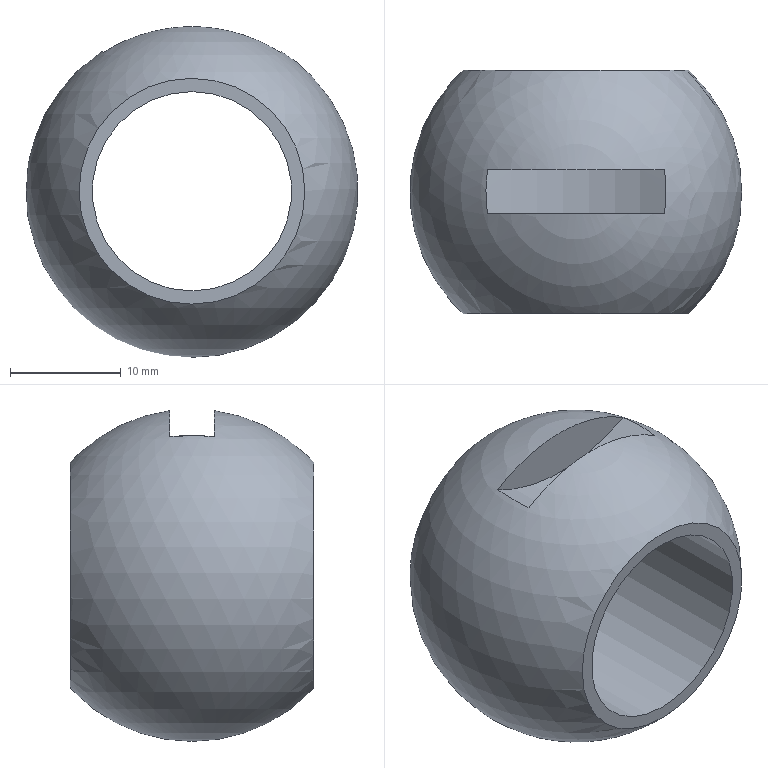Component | NX | VALVE_CORE | 1 solid | 7 faces | box 30 x 22 x 29.87 mm | volume 6970 mm3 | plane 4 | cylinder 2 | sphere 1 | commonest cylinder face diameters 18 x1 33.5 x1
STEP:
#1=CARTESIAN_POINT('',(0.,0.,0.));
#2=DIRECTION('',(0.,0.,1.));
#3=DIRECTION('',(1.,0.,0.));
#4=AXIS2_PLACEMENT_3D('',#1,#2,#3);
#5=CARTESIAN_POINT('',(-7.997,16.,31.532));
#6=VERTEX_POINT('',#5);
#7=CARTESIAN_POINT('',(-7.997,12.,31.532));
#8=VERTEX_POINT('',#7);
#9=CARTESIAN_POINT('',(-7.997,16.,31.532));
#10=CARTESIAN_POINT('',(-8.177,14.667,31.63));
#11=CARTESIAN_POINT('',(-8.177,13.333,31.63));
#12=CARTESIAN_POINT('',(-7.997,12.,31.532));
#13=B_SPLINE_CURVE_WITH_KNOTS('',3,(#9,#10,#11,#12),.UNSPECIFIED.,.F.,.F.,(4,4),(0.,1.),.PIECEWISE_BEZIER_KNOTS.);
#14=CARTESIAN_POINT('',(-0.,14.,19.));
#15=DIRECTION('',(0.,0.,1.));
#16=DIRECTION('',(1.,0.,-0.));
#17=AXIS2_PLACEMENT_3D('',#14,#15,#16);
#18=SPHERICAL_SURFACE('',#17,15.);
#19=CARTESIAN_POINT('',(2.897,0.989));
#20=CARTESIAN_POINT('',(2.904,0.9895));
#21=CARTESIAN_POINT('',(2.919,0.9906));
#22=CARTESIAN_POINT('',(2.941,0.992));
#23=CARTESIAN_POINT('',(2.963,0.9932));
#24=CARTESIAN_POINT('',(2.985,0.9943));
#25=CARTESIAN_POINT('',(3.008,0.9953));
#26=CARTESIAN_POINT('',(3.03,0.9961));
#27=CARTESIAN_POINT('',(3.052,0.9967));
#28=CARTESIAN_POINT('',(3.075,0.9972));
#29=CARTESIAN_POINT('',(3.097,0.9976));
#30=CARTESIAN_POINT('',(3.119,0.9978));
#31=CARTESIAN_POINT('',(3.142,0.9979));
#32=CARTESIAN_POINT('',(3.164,0.9978));
#33=CARTESIAN_POINT('',(3.186,0.9976));
#34=CARTESIAN_POINT('',(3.209,0.9972));
#35=CARTESIAN_POINT('',(3.231,0.9967));
#36=CARTESIAN_POINT('',(3.253,0.9961));
#37=CARTESIAN_POINT('',(3.276,0.9953));
#38=CARTESIAN_POINT('',(3.298,0.9943));
#39=CARTESIAN_POINT('',(3.32,0.9932));
#40=CARTESIAN_POINT('',(3.342,0.992));
#41=CARTESIAN_POINT('',(3.365,0.9906));
#42=CARTESIAN_POINT('',(3.379,0.9895));
#43=CARTESIAN_POINT('',(3.387,0.989));
#44=B_SPLINE_CURVE_WITH_KNOTS('',3,(#19,#20,#21,#22,#23,#24,#25,#26,#27,#28,#29,#30,#31,#32,#33,#34,#35,#36,#37,#38,#39,#40,#41,#42,#43),.UNSPECIFIED.,.F.,.F.,(4,1,1,1,1,1,1,1,1,1,1,1,1,1,1,1,1,1,1,1,1,1,4),(0.,0.04545,0.09091,0.1364,0.1818,0.2273,0.2727,0.3182,0.3636,0.4091,0.4545,0.5,0.5455,0.5909,0.6364,0.6818,0.7273,0.7727,0.8182,0.8636,0.9091,0.9545,1.),.QUASI_UNIFORM_KNOTS.);
#45=(GEOMETRIC_REPRESENTATION_CONTEXT(2)PARAMETRIC_REPRESENTATION_CONTEXT()REPRESENTATION_CONTEXT('',''));
#46=DEFINITIONAL_REPRESENTATION('',(#44),#45);
#47=PCURVE('',#18,#46);
#48=CARTESIAN_POINT('',(-0.,16.,46.25));
#49=DIRECTION('',(0.,-1.,0.));
#50=DIRECTION('',(0.,0.,-1.));
#51=AXIS2_PLACEMENT_3D('',#48,#49,#50);
#52=CYLINDRICAL_SURFACE('',#51,16.75);
#53=CARTESIAN_POINT('',(5.785,0.));
#54=CARTESIAN_POINT('',(5.785,0.06061));
#55=CARTESIAN_POINT('',(5.784,0.1818));
#56=CARTESIAN_POINT('',(5.782,0.3636));
#57=CARTESIAN_POINT('',(5.781,0.5455));
#58=CARTESIAN_POINT('',(5.78,0.7273));
#59=CARTESIAN_POINT('',(5.779,0.9091));
#60=CARTESIAN_POINT('',(5.778,1.091));
#61=CARTESIAN_POINT('',(5.777,1.273));
#62=CARTESIAN_POINT('',(5.777,1.455));
#63=CARTESIAN_POINT('',(5.777,1.636));
#64=CARTESIAN_POINT('',(5.776,1.818));
#65=CARTESIAN_POINT('',(5.776,2.));
#66=CARTESIAN_POINT('',(5.776,2.182));
#67=CARTESIAN_POINT('',(5.777,2.364));
#68=CARTESIAN_POINT('',(5.777,2.545));
#69=CARTESIAN_POINT('',(5.777,2.727));
#70=CARTESIAN_POINT('',(5.778,2.909));
#71=CARTESIAN_POINT('',(5.779,3.091));
#72=CARTESIAN_POINT('',(5.78,3.273));
#73=CARTESIAN_POINT('',(5.781,3.455));
#74=CARTESIAN_POINT('',(5.782,3.636));
#75=CARTESIAN_POINT('',(5.784,3.818));
#76=CARTESIAN_POINT('',(5.785,3.939));
#77=CARTESIAN_POINT('',(5.785,4.));
#78=B_SPLINE_CURVE_WITH_KNOTS('',3,(#53,#54,#55,#56,#57,#58,#59,#60,#61,#62,#63,#64,#65,#66,#67,#68,#69,#70,#71,#72,#73,#74,#75,#76,#77),.UNSPECIFIED.,.F.,.F.,(4,1,1,1,1,1,1,1,1,1,1,1,1,1,1,1,1,1,1,1,1,1,4),(0.,0.04545,0.09091,0.1364,0.1818,0.2273,0.2727,0.3182,0.3636,0.4091,0.4545,0.5,0.5455,0.5909,0.6364,0.6818,0.7273,0.7727,0.8182,0.8636,0.9091,0.9545,1.),.QUASI_UNIFORM_KNOTS.);
#79=(GEOMETRIC_REPRESENTATION_CONTEXT(2)PARAMETRIC_REPRESENTATION_CONTEXT()REPRESENTATION_CONTEXT('',''));
#80=DEFINITIONAL_REPRESENTATION('',(#78),#79);
#81=PCURVE('',#52,#80);
#82=SURFACE_CURVE('',#13,(#47,#81),.PCURVE_S1.);
#83=EDGE_CURVE('',#6,#8,#82,.T.);
#84=ORIENTED_EDGE('',*,*,#83,.F.);
#85=CARTESIAN_POINT('',(7.997,16.,31.532));
#86=VERTEX_POINT('',#85);
#87=CARTESIAN_POINT('',(-0.,16.,19.));
#88=DIRECTION('',(0.,1.,0.));
#89=DIRECTION('',(0.,0.,-1.));
#90=AXIS2_PLACEMENT_3D('',#87,#88,#89);
#91=CIRCLE('',#90,14.866);
#92=CARTESIAN_POINT('',(2.897,0.989));
#93=CARTESIAN_POINT('',(2.89,1.006));
#94=CARTESIAN_POINT('',(2.876,1.039));
#95=CARTESIAN_POINT('',(2.851,1.089));
#96=CARTESIAN_POINT('',(2.82,1.138));
#97=CARTESIAN_POINT('',(2.78,1.187));
#98=CARTESIAN_POINT('',(2.729,1.234));
#99=CARTESIAN_POINT('',(2.661,1.281));
#100=CARTESIAN_POINT('',(2.568,1.326));
#101=CARTESIAN_POINT('',(2.435,1.367));
#102=CARTESIAN_POINT('',(2.24,1.404));
#103=CARTESIAN_POINT('',(1.953,1.43));
#104=CARTESIAN_POINT('',(1.571,1.44));
#105=CARTESIAN_POINT('',(1.189,1.43));
#106=CARTESIAN_POINT('',(0.9016,1.404));
#107=CARTESIAN_POINT('',(0.7068,1.367));
#108=CARTESIAN_POINT('',(0.574,1.326));
#109=CARTESIAN_POINT('',(0.4808,1.281));
#110=CARTESIAN_POINT('',(0.4128,1.234));
#111=CARTESIAN_POINT('',(0.3616,1.187));
#112=CARTESIAN_POINT('',(0.322,1.138));
#113=CARTESIAN_POINT('',(0.2906,1.089));
#114=CARTESIAN_POINT('',(0.2653,1.039));
#115=CARTESIAN_POINT('',(0.2515,1.006));
#116=CARTESIAN_POINT('',(0.2451,0.989));
#117=B_SPLINE_CURVE_WITH_KNOTS('',3,(#92,#93,#94,#95,#96,#97,#98,#99,#100,#101,#102,#103,#104,#105,#106,#107,#108,#109,#110,#111,#112,#113,#114,#115,#116),.UNSPECIFIED.,.F.,.F.,(4,1,1,1,1,1,1,1,1,1,1,1,1,1,1,1,1,1,1,1,1,1,4),(2.574,2.625,2.677,2.729,2.78,2.832,2.883,2.935,2.987,3.038,3.09,3.142,3.193,3.245,3.296,3.348,3.4,3.451,3.503,3.555,3.606,3.658,3.71),.QUASI_UNIFORM_KNOTS.);
#118=(GEOMETRIC_REPRESENTATION_CONTEXT(2)PARAMETRIC_REPRESENTATION_CONTEXT()REPRESENTATION_CONTEXT('',''));
#119=DEFINITIONAL_REPRESENTATION('',(#117),#118);
#120=PCURVE('',#18,#119);
#121=CARTESIAN_POINT('',(-0.,16.,46.25));
#122=DIRECTION('',(0.,-1.,0.));
#123=DIRECTION('',(0.,0.,-1.));
#124=AXIS2_PLACEMENT_3D('',#121,#122,#123);
#125=PLANE('',#124);
#126=CARTESIAN_POINT('',(42.116,0.));
#127=CARTESIAN_POINT('',(42.116,-25.749));
#128=CARTESIAN_POINT('',(19.817,-12.874));
#129=CARTESIAN_POINT('',(-2.482,-0.));
#130=CARTESIAN_POINT('',(19.817,12.874));
#131=CARTESIAN_POINT('',(42.116,25.749));
#132=CARTESIAN_POINT('',(42.116,0.));
#133=(BOUNDED_CURVE()B_SPLINE_CURVE(2,(#126,#127,#128,#129,#130,#131,#132),.UNSPECIFIED.,.T.,.F.)B_SPLINE_CURVE_WITH_KNOTS((1,2,2,2,2,1),(-2.094,0.,2.094,4.189,6.283,8.378),.UNSPECIFIED.)CURVE()GEOMETRIC_REPRESENTATION_ITEM()RATIONAL_B_SPLINE_CURVE((1.,0.5,1.,0.5,1.,0.5,1.))REPRESENTATION_ITEM(''));
#134=(GEOMETRIC_REPRESENTATION_CONTEXT(2)PARAMETRIC_REPRESENTATION_CONTEXT()REPRESENTATION_CONTEXT('',''));
#135=DEFINITIONAL_REPRESENTATION('',(#133),#134);
#136=PCURVE('',#125,#135);
#137=SURFACE_CURVE('',#91,(#120,#136),.PCURVE_S1.);
#138=EDGE_CURVE('',#6,#86,#137,.T.);
#139=ORIENTED_EDGE('',*,*,#138,.T.);
#140=CARTESIAN_POINT('',(8.131,14.,31.605));
#141=VERTEX_POINT('',#140);
#142=CARTESIAN_POINT('',(7.997,12.,31.532));
#143=CARTESIAN_POINT('',(8.177,13.333,31.63));
#144=CARTESIAN_POINT('',(8.177,14.667,31.63));
#145=CARTESIAN_POINT('',(7.997,16.,31.532));
#146=B_SPLINE_CURVE_WITH_KNOTS('',3,(#142,#143,#144,#145),.UNSPECIFIED.,.F.,.F.,(4,4),(0.,1.),.PIECEWISE_BEZIER_KNOTS.);
#147=CARTESIAN_POINT('',(-0.2451,0.989));
#148=CARTESIAN_POINT('',(-0.2377,0.9895));
#149=CARTESIAN_POINT('',(-0.2229,0.9906));
#150=CARTESIAN_POINT('',(-0.2008,0.992));
#151=CARTESIAN_POINT('',(-0.1785,0.9932));
#152=CARTESIAN_POINT('',(-0.1563,0.9943));
#153=CARTESIAN_POINT('',(-0.134,0.9953));
#154=CARTESIAN_POINT('',(-0.1117,0.9961));
#155=CARTESIAN_POINT('',(-0.0894,0.9967));
#156=CARTESIAN_POINT('',(-0.06706,0.9972));
#157=CARTESIAN_POINT('',(-0.04471,0.9976));
#158=CARTESIAN_POINT('',(-0.02236,0.9978));
#159=CARTESIAN_POINT('',(0.,0.9979));
#160=CARTESIAN_POINT('',(0.02236,0.9978));
#161=CARTESIAN_POINT('',(0.04471,0.9976));
#162=CARTESIAN_POINT('',(0.06706,0.9972));
#163=CARTESIAN_POINT('',(0.0894,0.9967));
#164=CARTESIAN_POINT('',(0.1117,0.9961));
#165=CARTESIAN_POINT('',(0.134,0.9953));
#166=CARTESIAN_POINT('',(0.1563,0.9943));
#167=CARTESIAN_POINT('',(0.1785,0.9932));
#168=CARTESIAN_POINT('',(0.2008,0.992));
#169=CARTESIAN_POINT('',(0.2229,0.9906));
#170=CARTESIAN_POINT('',(0.2377,0.9895));
#171=CARTESIAN_POINT('',(0.2451,0.989));
#172=B_SPLINE_CURVE_WITH_KNOTS('',3,(#147,#148,#149,#150,#151,#152,#153,#154,#155,#156,#157,#158,#159,#160,#161,#162,#163,#164,#165,#166,#167,#168,#169,#170,#171),.UNSPECIFIED.,.F.,.F.,(4,1,1,1,1,1,1,1,1,1,1,1,1,1,1,1,1,1,1,1,1,1,4),(0.,0.04545,0.09091,0.1364,0.1818,0.2273,0.2727,0.3182,0.3636,0.4091,0.4545,0.5,0.5455,0.5909,0.6364,0.6818,0.7273,0.7727,0.8182,0.8636,0.9091,0.9545,1.),.QUASI_UNIFORM_KNOTS.);
#173=(GEOMETRIC_REPRESENTATION_CONTEXT(2)PARAMETRIC_REPRESENTATION_CONTEXT()REPRESENTATION_CONTEXT('',''));
#174=DEFINITIONAL_REPRESENTATION('',(#172),#173);
#175=PCURVE('',#18,#174);
#176=CARTESIAN_POINT('',(6.79,2.));
#177=CARTESIAN_POINT('',(6.781,0.));
#178=B_SPLINE_CURVE_WITH_KNOTS('',1,(#176,#177),.UNSPECIFIED.,.F.,.F.,(2,2),(0.5,1.),.PIECEWISE_BEZIER_KNOTS.);
#179=(GEOMETRIC_REPRESENTATION_CONTEXT(2)PARAMETRIC_REPRESENTATION_CONTEXT()REPRESENTATION_CONTEXT('',''));
#180=DEFINITIONAL_REPRESENTATION('',(#178),#179);
#181=PCURVE('',#52,#180);
#182=SURFACE_CURVE('',#146,(#175,#181),.PCURVE_S1.);
#183=EDGE_CURVE('',#141,#86,#182,.T.);
#184=ORIENTED_EDGE('',*,*,#183,.F.);
#185=CARTESIAN_POINT('',(-0.,14.,4.));
#186=VERTEX_POINT('',#185);
#187=CARTESIAN_POINT('',(0.,14.,4.));
#188=CARTESIAN_POINT('',(4.816,14.,4.));
#189=CARTESIAN_POINT('',(9.633,14.,5.767));
#190=CARTESIAN_POINT('',(13.692,14.,9.302));
#191=CARTESIAN_POINT('',(16.239,14.,14.217));
#192=CARTESIAN_POINT('',(16.763,14.,19.728));
#193=CARTESIAN_POINT('',(15.268,14.,24.898));
#194=CARTESIAN_POINT('',(12.179,14.,28.994));
#195=CARTESIAN_POINT('',(8.131,14.,31.605));
#196=B_SPLINE_CURVE_WITH_KNOTS('',8,(#187,#188,#189,#190,#191,#192,#193,#194,#195),.UNSPECIFIED.,.F.,.F.,(9,9),(-1.571,0.9979),.PIECEWISE_BEZIER_KNOTS.);
#197=CARTESIAN_POINT('',(0.,0.));
#198=DIRECTION('',(0.,1.));
#199=VECTOR('',#198,1.);
#200=LINE('',#197,#199);
#201=(GEOMETRIC_REPRESENTATION_CONTEXT(2)PARAMETRIC_REPRESENTATION_CONTEXT()REPRESENTATION_CONTEXT('',''));
#202=DEFINITIONAL_REPRESENTATION('',(#200),#201);
#203=PCURVE('',#18,#202);
#204=CARTESIAN_POINT('',(6.283,0.));
#205=DIRECTION('',(0.,1.));
#206=VECTOR('',#205,1.);
#207=LINE('',#204,#206);
#208=(GEOMETRIC_REPRESENTATION_CONTEXT(2)PARAMETRIC_REPRESENTATION_CONTEXT()REPRESENTATION_CONTEXT('',''));
#209=DEFINITIONAL_REPRESENTATION('',(#207),#208);
#210=PCURVE('',#18,#209);
#211=SEAM_CURVE('',#196,(#203,#210),.PCURVE_S1.);
#212=EDGE_CURVE('',#186,#141,#211,.T.);
#213=ORIENTED_EDGE('',*,*,#212,.F.);
#214=ORIENTED_EDGE('',*,*,#212,.T.);
#215=CARTESIAN_POINT('',(7.997,12.,31.532));
#216=VERTEX_POINT('',#215);
#217=CARTESIAN_POINT('',(7.997,12.,31.532));
#218=CARTESIAN_POINT('',(8.177,13.333,31.63));
#219=CARTESIAN_POINT('',(8.177,14.667,31.63));
#220=CARTESIAN_POINT('',(7.997,16.,31.532));
#221=B_SPLINE_CURVE_WITH_KNOTS('',3,(#217,#218,#219,#220),.UNSPECIFIED.,.F.,.F.,(4,4),(0.,1.),.PIECEWISE_BEZIER_KNOTS.);
#222=CARTESIAN_POINT('',(6.038,0.989));
#223=CARTESIAN_POINT('',(6.045,0.9895));
#224=CARTESIAN_POINT('',(6.06,0.9906));
#225=CARTESIAN_POINT('',(6.082,0.992));
#226=CARTESIAN_POINT('',(6.105,0.9932));
#227=CARTESIAN_POINT('',(6.127,0.9943));
#228=CARTESIAN_POINT('',(6.149,0.9953));
#229=CARTESIAN_POINT('',(6.171,0.9961));
#230=CARTESIAN_POINT('',(6.194,0.9967));
#231=CARTESIAN_POINT('',(6.216,0.9972));
#232=CARTESIAN_POINT('',(6.238,0.9976));
#233=CARTESIAN_POINT('',(6.261,0.9978));
#234=CARTESIAN_POINT('',(6.283,0.9979));
#235=CARTESIAN_POINT('',(6.306,0.9978));
#236=CARTESIAN_POINT('',(6.328,0.9976));
#237=CARTESIAN_POINT('',(6.35,0.9972));
#238=CARTESIAN_POINT('',(6.373,0.9967));
#239=CARTESIAN_POINT('',(6.395,0.9961));
#240=CARTESIAN_POINT('',(6.417,0.9953));
#241=CARTESIAN_POINT('',(6.439,0.9943));
#242=CARTESIAN_POINT('',(6.462,0.9932));
#243=CARTESIAN_POINT('',(6.484,0.992));
#244=CARTESIAN_POINT('',(6.506,0.9906));
#245=CARTESIAN_POINT('',(6.521,0.9895));
#246=CARTESIAN_POINT('',(6.528,0.989));
#247=B_SPLINE_CURVE_WITH_KNOTS('',3,(#222,#223,#224,#225,#226,#227,#228,#229,#230,#231,#232,#233,#234,#235,#236,#237,#238,#239,#240,#241,#242,#243,#244,#245,#246),.UNSPECIFIED.,.F.,.F.,(4,1,1,1,1,1,1,1,1,1,1,1,1,1,1,1,1,1,1,1,1,1,4),(0.,0.04545,0.09091,0.1364,0.1818,0.2273,0.2727,0.3182,0.3636,0.4091,0.4545,0.5,0.5455,0.5909,0.6364,0.6818,0.7273,0.7727,0.8182,0.8636,0.9091,0.9545,1.),.QUASI_UNIFORM_KNOTS.);
#248=(GEOMETRIC_REPRESENTATION_CONTEXT(2)PARAMETRIC_REPRESENTATION_CONTEXT()REPRESENTATION_CONTEXT('',''));
#249=DEFINITIONAL_REPRESENTATION('',(#247),#248);
#250=PCURVE('',#18,#249);
#251=CARTESIAN_POINT('',(6.781,4.));
#252=CARTESIAN_POINT('',(6.79,2.));
#253=B_SPLINE_CURVE_WITH_KNOTS('',1,(#251,#252),.UNSPECIFIED.,.F.,.F.,(2,2),(0.,0.5),.PIECEWISE_BEZIER_KNOTS.);
#254=(GEOMETRIC_REPRESENTATION_CONTEXT(2)PARAMETRIC_REPRESENTATION_CONTEXT()REPRESENTATION_CONTEXT('',''));
#255=DEFINITIONAL_REPRESENTATION('',(#253),#254);
#256=PCURVE('',#52,#255);
#257=SURFACE_CURVE('',#221,(#250,#256),.PCURVE_S1.);
#258=EDGE_CURVE('',#216,#141,#257,.T.);
#259=ORIENTED_EDGE('',*,*,#258,.F.);
#260=CARTESIAN_POINT('',(-0.,12.,19.));
#261=DIRECTION('',(0.,1.,0.));
#262=DIRECTION('',(0.,0.,-1.));
#263=AXIS2_PLACEMENT_3D('',#260,#261,#262);
#264=CIRCLE('',#263,14.866);
#265=CARTESIAN_POINT('',(3.387,0.989));
#266=CARTESIAN_POINT('',(3.393,1.006));
#267=CARTESIAN_POINT('',(3.407,1.039));
#268=CARTESIAN_POINT('',(3.432,1.089));
#269=CARTESIAN_POINT('',(3.464,1.138));
#270=CARTESIAN_POINT('',(3.503,1.187));
#271=CARTESIAN_POINT('',(3.554,1.234));
#272=CARTESIAN_POINT('',(3.622,1.281));
#273=CARTESIAN_POINT('',(3.716,1.326));
#274=CARTESIAN_POINT('',(3.848,1.367));
#275=CARTESIAN_POINT('',(4.043,1.404));
#276=CARTESIAN_POINT('',(4.33,1.43));
#277=CARTESIAN_POINT('',(4.712,1.44));
#278=CARTESIAN_POINT('',(5.095,1.43));
#279=CARTESIAN_POINT('',(5.382,1.404));
#280=CARTESIAN_POINT('',(5.576,1.367));
#281=CARTESIAN_POINT('',(5.709,1.326));
#282=CARTESIAN_POINT('',(5.802,1.281));
#283=CARTESIAN_POINT('',(5.87,1.234));
#284=CARTESIAN_POINT('',(5.922,1.187));
#285=CARTESIAN_POINT('',(5.961,1.138));
#286=CARTESIAN_POINT('',(5.993,1.089));
#287=CARTESIAN_POINT('',(6.018,1.039));
#288=CARTESIAN_POINT('',(6.032,1.006));
#289=CARTESIAN_POINT('',(6.038,0.989));
#290=B_SPLINE_CURVE_WITH_KNOTS('',3,(#265,#266,#267,#268,#269,#270,#271,#272,#273,#274,#275,#276,#277,#278,#279,#280,#281,#282,#283,#284,#285,#286,#287,#288,#289),.UNSPECIFIED.,.F.,.F.,(4,1,1,1,1,1,1,1,1,1,1,1,1,1,1,1,1,1,1,1,1,1,4),(2.574,2.625,2.677,2.729,2.78,2.832,2.883,2.935,2.987,3.038,3.09,3.142,3.193,3.245,3.296,3.348,3.4,3.451,3.503,3.555,3.606,3.658,3.71),.QUASI_UNIFORM_KNOTS.);
#291=(GEOMETRIC_REPRESENTATION_CONTEXT(2)PARAMETRIC_REPRESENTATION_CONTEXT()REPRESENTATION_CONTEXT('',''));
#292=DEFINITIONAL_REPRESENTATION('',(#290),#291);
#293=PCURVE('',#18,#292);
#294=CARTESIAN_POINT('',(-0.,12.,46.25));
#295=DIRECTION('',(0.,-1.,0.));
#296=DIRECTION('',(0.,0.,-1.));
#297=AXIS2_PLACEMENT_3D('',#294,#295,#296);
#298=PLANE('',#297);
#299=CARTESIAN_POINT('',(42.116,0.));
#300=CARTESIAN_POINT('',(42.116,-25.749));
#301=CARTESIAN_POINT('',(19.817,-12.874));
#302=CARTESIAN_POINT('',(-2.482,-0.));
#303=CARTESIAN_POINT('',(19.817,12.874));
#304=CARTESIAN_POINT('',(42.116,25.749));
#305=CARTESIAN_POINT('',(42.116,0.));
#306=(BOUNDED_CURVE()B_SPLINE_CURVE(2,(#299,#300,#301,#302,#303,#304,#305),.UNSPECIFIED.,.T.,.F.)B_SPLINE_CURVE_WITH_KNOTS((1,2,2,2,2,1),(-2.094,0.,2.094,4.189,6.283,8.378),.UNSPECIFIED.)CURVE()GEOMETRIC_REPRESENTATION_ITEM()RATIONAL_B_SPLINE_CURVE((1.,0.5,1.,0.5,1.,0.5,1.))REPRESENTATION_ITEM(''));
#307=(GEOMETRIC_REPRESENTATION_CONTEXT(2)PARAMETRIC_REPRESENTATION_CONTEXT()REPRESENTATION_CONTEXT('',''));
#308=DEFINITIONAL_REPRESENTATION('',(#306),#307);
#309=PCURVE('',#298,#308);
#310=SURFACE_CURVE('',#264,(#293,#309),.PCURVE_S1.);
#311=EDGE_CURVE('',#8,#216,#310,.T.);
#312=ORIENTED_EDGE('',*,*,#311,.F.);
#313=EDGE_LOOP('',(#84,#139,#184,#213,#214,#259,#312));
#314=FACE_BOUND('',#313,.T.);
#315=CARTESIAN_POINT('',(-0.,25.,29.198));
#316=VERTEX_POINT('',#315);
#317=CARTESIAN_POINT('',(-0.,25.,19.));
#318=DIRECTION('',(0.,-1.,0.));
#319=DIRECTION('',(0.,0.,1.));
#320=AXIS2_PLACEMENT_3D('',#317,#318,#319);
#321=CIRCLE('',#320,10.198);
#322=CARTESIAN_POINT('',(1.571,0.7476));
#323=CARTESIAN_POINT('',(1.662,0.7482));
#324=CARTESIAN_POINT('',(1.834,0.7215));
#325=CARTESIAN_POINT('',(2.047,0.6165));
#326=CARTESIAN_POINT('',(2.191,0.4659));
#327=CARTESIAN_POINT('',(2.279,0.2886));
#328=CARTESIAN_POINT('',(2.32,0.09761));
#329=CARTESIAN_POINT('',(2.32,-0.09761));
#330=CARTESIAN_POINT('',(2.279,-0.2886));
#331=CARTESIAN_POINT('',(2.192,-0.4659));
#332=CARTESIAN_POINT('',(2.046,-0.6164));
#333=CARTESIAN_POINT('',(1.835,-0.7218));
#334=CARTESIAN_POINT('',(1.571,-0.7605));
#335=CARTESIAN_POINT('',(1.306,-0.7218));
#336=CARTESIAN_POINT('',(1.095,-0.6164));
#337=CARTESIAN_POINT('',(0.9501,-0.4659));
#338=CARTESIAN_POINT('',(0.8624,-0.2886));
#339=CARTESIAN_POINT('',(0.8215,-0.09761));
#340=CARTESIAN_POINT('',(0.8215,0.09761));
#341=CARTESIAN_POINT('',(0.8624,0.2886));
#342=CARTESIAN_POINT('',(0.9502,0.4659));
#343=CARTESIAN_POINT('',(1.095,0.6165));
#344=CARTESIAN_POINT('',(1.308,0.7215));
#345=CARTESIAN_POINT('',(1.48,0.7482));
#346=CARTESIAN_POINT('',(1.571,0.7476));
#347=B_SPLINE_CURVE_WITH_KNOTS('',3,(#322,#323,#324,#325,#326,#327,#328,#329,#330,#331,#332,#333,#334,#335,#336,#337,#338,#339,#340,#341,#342,#343,#344,#345,#346),.UNSPECIFIED.,.F.,.F.,(4,1,1,1,1,1,1,1,1,1,1,1,1,1,1,1,1,1,1,1,1,1,4),(0.,0.2856,0.5712,0.8568,1.142,1.428,1.714,1.999,2.285,2.57,2.856,3.142,3.427,3.713,3.998,4.284,4.57,4.855,5.141,5.426,5.712,5.998,6.283),.QUASI_UNIFORM_KNOTS.);
#348=(GEOMETRIC_REPRESENTATION_CONTEXT(2)PARAMETRIC_REPRESENTATION_CONTEXT()REPRESENTATION_CONTEXT('',''));
#349=DEFINITIONAL_REPRESENTATION('',(#347),#348);
#350=PCURVE('',#18,#349);
#351=CARTESIAN_POINT('',(-0.,25.,19.));
#352=DIRECTION('',(0.,1.,0.));
#353=DIRECTION('',(0.,0.,1.));
#354=AXIS2_PLACEMENT_3D('',#351,#352,#353);
#355=PLANE('',#354);
#356=CARTESIAN_POINT('',(10.198,0.));
#357=CARTESIAN_POINT('',(10.198,-17.664));
#358=CARTESIAN_POINT('',(-5.099,-8.832));
#359=CARTESIAN_POINT('',(-20.396,-0.));
#360=CARTESIAN_POINT('',(-5.099,8.832));
#361=CARTESIAN_POINT('',(10.198,17.664));
#362=CARTESIAN_POINT('',(10.198,0.));
#363=(BOUNDED_CURVE()B_SPLINE_CURVE(2,(#356,#357,#358,#359,#360,#361,#362),.UNSPECIFIED.,.T.,.F.)B_SPLINE_CURVE_WITH_KNOTS((1,2,2,2,2,1),(-2.094,0.,2.094,4.189,6.283,8.378),.UNSPECIFIED.)CURVE()GEOMETRIC_REPRESENTATION_ITEM()RATIONAL_B_SPLINE_CURVE((1.,0.5,1.,0.5,1.,0.5,1.))REPRESENTATION_ITEM(''));
#364=(GEOMETRIC_REPRESENTATION_CONTEXT(2)PARAMETRIC_REPRESENTATION_CONTEXT()REPRESENTATION_CONTEXT('',''));
#365=DEFINITIONAL_REPRESENTATION('',(#363),#364);
#366=PCURVE('',#355,#365);
#367=SURFACE_CURVE('',#321,(#350,#366),.PCURVE_S1.);
#368=EDGE_CURVE('',#316,#316,#367,.T.);
#369=ORIENTED_EDGE('',*,*,#368,.T.);
#370=EDGE_LOOP('',(#369));
#371=FACE_BOUND('',#370,.T.);
#372=CARTESIAN_POINT('',(-0.,3.,8.802));
#373=VERTEX_POINT('',#372);
#374=CARTESIAN_POINT('',(-0.,3.,19.));
#375=DIRECTION('',(0.,1.,0.));
#376=DIRECTION('',(0.,0.,-1.));
#377=AXIS2_PLACEMENT_3D('',#374,#375,#376);
#378=CIRCLE('',#377,10.198);
#379=CARTESIAN_POINT('',(4.712,-0.7476));
#380=CARTESIAN_POINT('',(4.621,-0.7482));
#381=CARTESIAN_POINT('',(4.449,-0.7215));
#382=CARTESIAN_POINT('',(4.236,-0.6165));
#383=CARTESIAN_POINT('',(4.092,-0.4659));
#384=CARTESIAN_POINT('',(4.004,-0.2886));
#385=CARTESIAN_POINT('',(3.963,-0.09761));
#386=CARTESIAN_POINT('',(3.963,0.09761));
#387=CARTESIAN_POINT('',(4.004,0.2886));
#388=CARTESIAN_POINT('',(4.092,0.4659));
#389=CARTESIAN_POINT('',(4.237,0.6164));
#390=CARTESIAN_POINT('',(4.448,0.7218));
#391=CARTESIAN_POINT('',(4.712,0.7605));
#392=CARTESIAN_POINT('',(4.977,0.7218));
#393=CARTESIAN_POINT('',(5.188,0.6164));
#394=CARTESIAN_POINT('',(5.333,0.4659));
#395=CARTESIAN_POINT('',(5.421,0.2886));
#396=CARTESIAN_POINT('',(5.462,0.09761));
#397=CARTESIAN_POINT('',(5.462,-0.09761));
#398=CARTESIAN_POINT('',(5.421,-0.2886));
#399=CARTESIAN_POINT('',(5.333,-0.4659));
#400=CARTESIAN_POINT('',(5.188,-0.6165));
#401=CARTESIAN_POINT('',(4.975,-0.7215));
#402=CARTESIAN_POINT('',(4.803,-0.7482));
#403=CARTESIAN_POINT('',(4.712,-0.7476));
#404=B_SPLINE_CURVE_WITH_KNOTS('',3,(#379,#380,#381,#382,#383,#384,#385,#386,#387,#388,#389,#390,#391,#392,#393,#394,#395,#396,#397,#398,#399,#400,#401,#402,#403),.UNSPECIFIED.,.T.,.F.,(4,1,1,1,1,1,1,1,1,1,1,1,1,1,1,1,1,1,1,1,1,1,4),(0.,0.2856,0.5712,0.8568,1.142,1.428,1.714,1.999,2.285,2.57,2.856,3.142,3.427,3.713,3.998,4.284,4.57,4.855,5.141,5.426,5.712,5.998,6.283),.QUASI_UNIFORM_KNOTS.);
#405=(GEOMETRIC_REPRESENTATION_CONTEXT(2)PARAMETRIC_REPRESENTATION_CONTEXT()REPRESENTATION_CONTEXT('',''));
#406=DEFINITIONAL_REPRESENTATION('',(#404),#405);
#407=PCURVE('',#18,#406);
#408=CARTESIAN_POINT('',(-0.,3.,19.));
#409=DIRECTION('',(0.,-1.,0.));
#410=DIRECTION('',(0.,0.,-1.));
#411=AXIS2_PLACEMENT_3D('',#408,#409,#410);
#412=PLANE('',#411);
#413=CARTESIAN_POINT('',(10.198,0.));
#414=CARTESIAN_POINT('',(10.198,-17.664));
#415=CARTESIAN_POINT('',(-5.099,-8.832));
#416=CARTESIAN_POINT('',(-20.396,-0.));
#417=CARTESIAN_POINT('',(-5.099,8.832));
#418=CARTESIAN_POINT('',(10.198,17.664));
#419=CARTESIAN_POINT('',(10.198,0.));
#420=(BOUNDED_CURVE()B_SPLINE_CURVE(2,(#413,#414,#415,#416,#417,#418,#419),.UNSPECIFIED.,.T.,.F.)B_SPLINE_CURVE_WITH_KNOTS((1,2,2,2,2,1),(-2.094,0.,2.094,4.189,6.283,8.378),.UNSPECIFIED.)CURVE()GEOMETRIC_REPRESENTATION_ITEM()RATIONAL_B_SPLINE_CURVE((1.,0.5,1.,0.5,1.,0.5,1.))REPRESENTATION_ITEM(''));
#421=(GEOMETRIC_REPRESENTATION_CONTEXT(2)PARAMETRIC_REPRESENTATION_CONTEXT()REPRESENTATION_CONTEXT('',''));
#422=DEFINITIONAL_REPRESENTATION('',(#420),#421);
#423=PCURVE('',#412,#422);
#424=SURFACE_CURVE('',#378,(#407,#423),.PCURVE_S1.);
#425=EDGE_CURVE('',#373,#373,#424,.T.);
#426=ORIENTED_EDGE('',*,*,#425,.T.);
#427=EDGE_LOOP('',(#426));
#428=FACE_BOUND('',#427,.T.);
#429=ADVANCED_FACE('',(#314,#371,#428),#18,.T.);
#430=CARTESIAN_POINT('',(-0.,25.,28.));
#431=VERTEX_POINT('',#430);
#432=CARTESIAN_POINT('',(-0.,25.,19.));
#433=DIRECTION('',(0.,1.,0.));
#434=DIRECTION('',(0.,0.,1.));
#435=AXIS2_PLACEMENT_3D('',#432,#433,#434);
#436=CIRCLE('',#435,9.);
#437=CARTESIAN_POINT('',(0.,0.));
#438=DIRECTION('',(1.,0.));
#439=AXIS2_PLACEMENT_2D('',#437,#438);
#440=CIRCLE('',#439,9.);
#441=(GEOMETRIC_REPRESENTATION_CONTEXT(2)PARAMETRIC_REPRESENTATION_CONTEXT()REPRESENTATION_CONTEXT('',''));
#442=DEFINITIONAL_REPRESENTATION('',(#440),#441);
#443=PCURVE('',#355,#442);
#444=CARTESIAN_POINT('',(-0.,3.,19.));
#445=DIRECTION('',(0.,1.,0.));
#446=DIRECTION('',(0.,0.,1.));
#447=AXIS2_PLACEMENT_3D('',#444,#445,#446);
#448=CYLINDRICAL_SURFACE('',#447,9.);
#449=CARTESIAN_POINT('',(0.,22.));
#450=DIRECTION('',(1.,0.));
#451=VECTOR('',#450,1.);
#452=LINE('',#449,#451);
#453=(GEOMETRIC_REPRESENTATION_CONTEXT(2)PARAMETRIC_REPRESENTATION_CONTEXT()REPRESENTATION_CONTEXT('',''));
#454=DEFINITIONAL_REPRESENTATION('',(#452),#453);
#455=PCURVE('',#448,#454);
#456=SURFACE_CURVE('',#436,(#443,#455),.PCURVE_S1.);
#457=EDGE_CURVE('',#431,#431,#456,.T.);
#458=ORIENTED_EDGE('',*,*,#457,.F.);
#459=EDGE_LOOP('',(#458));
#460=FACE_BOUND('',#459,.T.);
#461=ORIENTED_EDGE('',*,*,#368,.F.);
#462=EDGE_LOOP('',(#461));
#463=FACE_BOUND('',#462,.T.);
#464=ADVANCED_FACE('',(#460,#463),#355,.T.);
#465=CARTESIAN_POINT('',(-0.,3.,28.));
#466=VERTEX_POINT('',#465);
#467=CARTESIAN_POINT('',(-0.,3.,19.));
#468=DIRECTION('',(0.,1.,0.));
#469=DIRECTION('',(0.,0.,1.));
#470=AXIS2_PLACEMENT_3D('',#467,#468,#469);
#471=CIRCLE('',#470,9.);
#472=CARTESIAN_POINT('',(-9.,0.));
#473=CARTESIAN_POINT('',(-9.,15.588));
#474=CARTESIAN_POINT('',(4.5,7.794));
#475=CARTESIAN_POINT('',(18.,0.));
#476=CARTESIAN_POINT('',(4.5,-7.794));
#477=CARTESIAN_POINT('',(-9.,-15.588));
#478=CARTESIAN_POINT('',(-9.,0.));
#479=(BOUNDED_CURVE()B_SPLINE_CURVE(2,(#472,#473,#474,#475,#476,#477,#478),.UNSPECIFIED.,.T.,.F.)B_SPLINE_CURVE_WITH_KNOTS((1,2,2,2,2,1),(-2.094,0.,2.094,4.189,6.283,8.378),.UNSPECIFIED.)CURVE()GEOMETRIC_REPRESENTATION_ITEM()RATIONAL_B_SPLINE_CURVE((1.,0.5,1.,0.5,1.,0.5,1.))REPRESENTATION_ITEM(''));
#480=(GEOMETRIC_REPRESENTATION_CONTEXT(2)PARAMETRIC_REPRESENTATION_CONTEXT()REPRESENTATION_CONTEXT('',''));
#481=DEFINITIONAL_REPRESENTATION('',(#479),#480);
#482=PCURVE('',#412,#481);
#483=CARTESIAN_POINT('',(0.,0.));
#484=DIRECTION('',(1.,0.));
#485=VECTOR('',#484,1.);
#486=LINE('',#483,#485);
#487=(GEOMETRIC_REPRESENTATION_CONTEXT(2)PARAMETRIC_REPRESENTATION_CONTEXT()REPRESENTATION_CONTEXT('',''));
#488=DEFINITIONAL_REPRESENTATION('',(#486),#487);
#489=PCURVE('',#448,#488);
#490=SURFACE_CURVE('',#471,(#482,#489),.PCURVE_S1.);
#491=EDGE_CURVE('',#466,#466,#490,.T.);
#492=ORIENTED_EDGE('',*,*,#491,.T.);
#493=EDGE_LOOP('',(#492));
#494=FACE_BOUND('',#493,.T.);
#495=ORIENTED_EDGE('',*,*,#425,.F.);
#496=EDGE_LOOP('',(#495));
#497=FACE_BOUND('',#496,.T.);
#498=ADVANCED_FACE('',(#494,#497),#412,.T.);
#499=ORIENTED_EDGE('',*,*,#457,.F.);
#500=CARTESIAN_POINT('',(-0.,3.,28.));
#501=CARTESIAN_POINT('',(-0.,25.,28.));
#502=B_SPLINE_CURVE_WITH_KNOTS('',1,(#500,#501),.UNSPECIFIED.,.F.,.F.,(2,2),(0.,22.),.PIECEWISE_BEZIER_KNOTS.);
#503=CARTESIAN_POINT('',(0.,0.));
#504=DIRECTION('',(0.,1.));
#505=VECTOR('',#504,1.);
#506=LINE('',#503,#505);
#507=(GEOMETRIC_REPRESENTATION_CONTEXT(2)PARAMETRIC_REPRESENTATION_CONTEXT()REPRESENTATION_CONTEXT('',''));
#508=DEFINITIONAL_REPRESENTATION('',(#506),#507);
#509=PCURVE('',#448,#508);
#510=CARTESIAN_POINT('',(6.283,0.));
#511=DIRECTION('',(0.,1.));
#512=VECTOR('',#511,1.);
#513=LINE('',#510,#512);
#514=(GEOMETRIC_REPRESENTATION_CONTEXT(2)PARAMETRIC_REPRESENTATION_CONTEXT()REPRESENTATION_CONTEXT('',''));
#515=DEFINITIONAL_REPRESENTATION('',(#513),#514);
#516=PCURVE('',#448,#515);
#517=SEAM_CURVE('',#502,(#509,#516),.PCURVE_S1.);
#518=EDGE_CURVE('',#466,#431,#517,.T.);
#519=ORIENTED_EDGE('',*,*,#518,.F.);
#520=ORIENTED_EDGE('',*,*,#491,.T.);
#521=ORIENTED_EDGE('',*,*,#518,.T.);
#522=EDGE_LOOP('',(#499,#519,#520,#521));
#523=FACE_BOUND('',#522,.F.);
#524=ADVANCED_FACE('',(#523),#448,.F.);
#525=CARTESIAN_POINT('',(-0.,16.,46.25));
#526=DIRECTION('',(0.,1.,0.));
#527=DIRECTION('',(1.,0.,0.));
#528=AXIS2_PLACEMENT_3D('',#525,#526,#527);
#529=CIRCLE('',#528,16.75);
#530=CARTESIAN_POINT('',(7.854,0.));
#531=DIRECTION('',(-1.,0.));
#532=VECTOR('',#531,1.);
#533=LINE('',#530,#532);
#534=(GEOMETRIC_REPRESENTATION_CONTEXT(2)PARAMETRIC_REPRESENTATION_CONTEXT()REPRESENTATION_CONTEXT('',''));
#535=DEFINITIONAL_REPRESENTATION('',(#533),#534);
#536=PCURVE('',#52,#535);
#537=CARTESIAN_POINT('',(0.,16.75));
#538=CARTESIAN_POINT('',(29.012,16.75));
#539=CARTESIAN_POINT('',(14.506,-8.375));
#540=CARTESIAN_POINT('',(0.,-33.5));
#541=CARTESIAN_POINT('',(-14.506,-8.375));
#542=CARTESIAN_POINT('',(-29.012,16.75));
#543=CARTESIAN_POINT('',(0.,16.75));
#544=(BOUNDED_CURVE()B_SPLINE_CURVE(2,(#537,#538,#539,#540,#541,#542,#543),.UNSPECIFIED.,.T.,.F.)B_SPLINE_CURVE_WITH_KNOTS((1,2,2,2,2,1),(-2.094,0.,2.094,4.189,6.283,8.378),.UNSPECIFIED.)CURVE()GEOMETRIC_REPRESENTATION_ITEM()RATIONAL_B_SPLINE_CURVE((1.,0.5,1.,0.5,1.,0.5,1.))REPRESENTATION_ITEM(''));
#545=(GEOMETRIC_REPRESENTATION_CONTEXT(2)PARAMETRIC_REPRESENTATION_CONTEXT()REPRESENTATION_CONTEXT('',''));
#546=DEFINITIONAL_REPRESENTATION('',(#544),#545);
#547=PCURVE('',#125,#546);
#548=SURFACE_CURVE('',#529,(#536,#547),.PCURVE_S1.);
#549=EDGE_CURVE('',#86,#6,#548,.T.);
#550=ORIENTED_EDGE('',*,*,#549,.F.);
#551=ORIENTED_EDGE('',*,*,#183,.F.);
#552=ORIENTED_EDGE('',*,*,#258,.F.);
#553=CARTESIAN_POINT('',(-0.,12.,46.25));
#554=DIRECTION('',(0.,1.,0.));
#555=DIRECTION('',(1.,0.,0.));
#556=AXIS2_PLACEMENT_3D('',#553,#554,#555);
#557=CIRCLE('',#556,16.75);
#558=CARTESIAN_POINT('',(7.854,4.));
#559=DIRECTION('',(-1.,0.));
#560=VECTOR('',#559,1.);
#561=LINE('',#558,#560);
#562=(GEOMETRIC_REPRESENTATION_CONTEXT(2)PARAMETRIC_REPRESENTATION_CONTEXT()REPRESENTATION_CONTEXT('',''));
#563=DEFINITIONAL_REPRESENTATION('',(#561),#562);
#564=PCURVE('',#52,#563);
#565=CARTESIAN_POINT('',(0.,16.75));
#566=CARTESIAN_POINT('',(29.012,16.75));
#567=CARTESIAN_POINT('',(14.506,-8.375));
#568=CARTESIAN_POINT('',(0.,-33.5));
#569=CARTESIAN_POINT('',(-14.506,-8.375));
#570=CARTESIAN_POINT('',(-29.012,16.75));
#571=CARTESIAN_POINT('',(0.,16.75));
#572=(BOUNDED_CURVE()B_SPLINE_CURVE(2,(#565,#566,#567,#568,#569,#570,#571),.UNSPECIFIED.,.T.,.F.)B_SPLINE_CURVE_WITH_KNOTS((1,2,2,2,2,1),(-2.094,0.,2.094,4.189,6.283,8.378),.UNSPECIFIED.)CURVE()GEOMETRIC_REPRESENTATION_ITEM()RATIONAL_B_SPLINE_CURVE((1.,0.5,1.,0.5,1.,0.5,1.))REPRESENTATION_ITEM(''));
#573=(GEOMETRIC_REPRESENTATION_CONTEXT(2)PARAMETRIC_REPRESENTATION_CONTEXT()REPRESENTATION_CONTEXT('',''));
#574=DEFINITIONAL_REPRESENTATION('',(#572),#573);
#575=PCURVE('',#298,#574);
#576=SURFACE_CURVE('',#557,(#564,#575),.PCURVE_S1.);
#577=EDGE_CURVE('',#216,#8,#576,.T.);
#578=ORIENTED_EDGE('',*,*,#577,.T.);
#579=ORIENTED_EDGE('',*,*,#83,.F.);
#580=EDGE_LOOP('',(#550,#551,#552,#578,#579));
#581=FACE_BOUND('',#580,.F.);
#582=ADVANCED_FACE('',(#581),#52,.F.);
#583=ORIENTED_EDGE('',*,*,#549,.F.);
#584=ORIENTED_EDGE('',*,*,#138,.F.);
#585=EDGE_LOOP('',(#583,#584));
#586=FACE_BOUND('',#585,.T.);
#587=ADVANCED_FACE('',(#586),#125,.T.);
#588=ORIENTED_EDGE('',*,*,#311,.T.);
#589=ORIENTED_EDGE('',*,*,#577,.T.);
#590=EDGE_LOOP('',(#588,#589));
#591=FACE_BOUND('',#590,.T.);
#592=ADVANCED_FACE('',(#591),#298,.F.);
#593=CLOSED_SHELL('',(#429,#464,#498,#524,#582,#587,#592));
#594=MANIFOLD_SOLID_BREP('',#593);
#595=(LENGTH_UNIT()NAMED_UNIT(*)SI_UNIT(.MILLI.,.METRE.));
#596=UNCERTAINTY_MEASURE_WITH_UNIT(LENGTH_MEASURE(0.01),#595,'','');
#597=(NAMED_UNIT(*)PLANE_ANGLE_UNIT()SI_UNIT($,.RADIAN.));
#598=(NAMED_UNIT(*)SI_UNIT($,.STERADIAN.)SOLID_ANGLE_UNIT());
#599=(GEOMETRIC_REPRESENTATION_CONTEXT(3)GLOBAL_UNCERTAINTY_ASSIGNED_CONTEXT((#596))GLOBAL_UNIT_ASSIGNED_CONTEXT((#595,#597,#598))REPRESENTATION_CONTEXT('',''));
#600=ADVANCED_BREP_SHAPE_REPRESENTATION('',(#4,#594),#599);